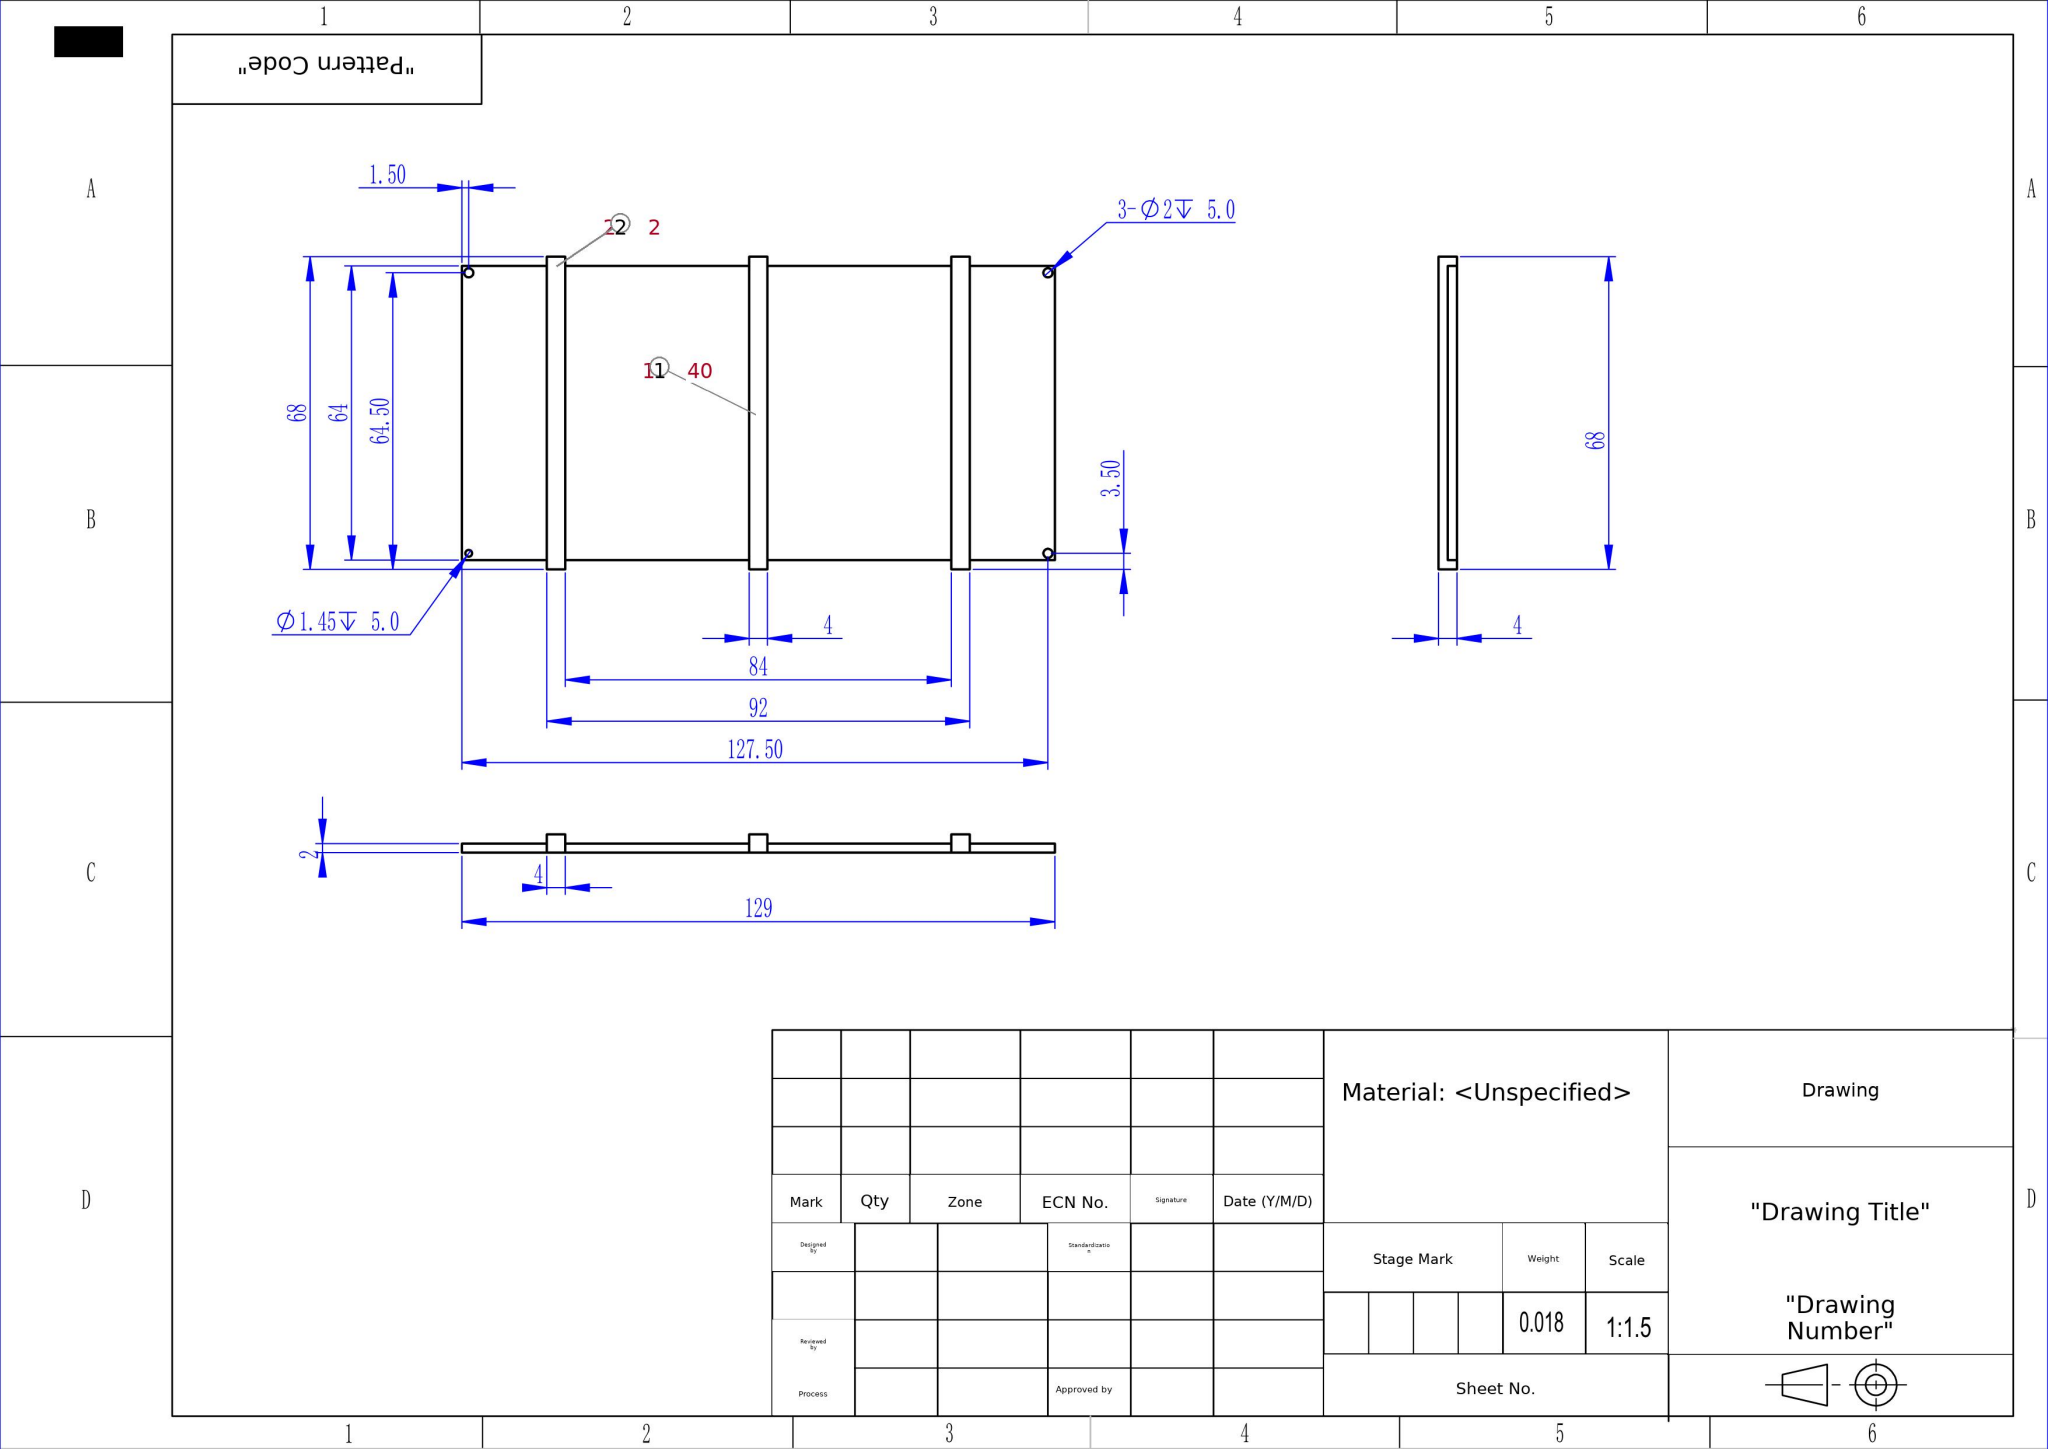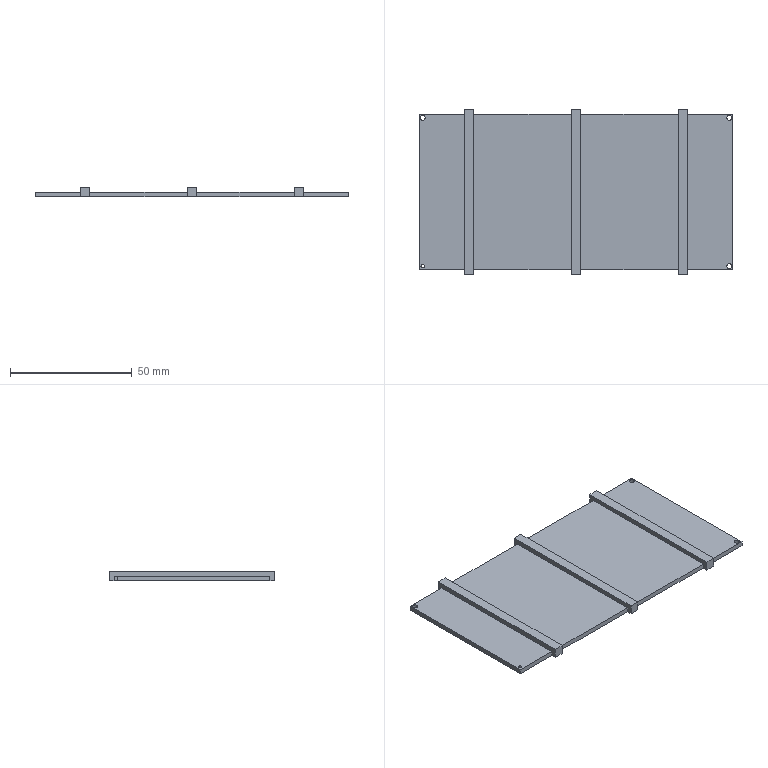Part | SolidWorks | mm | 1 solid | 38 faces | box 129 x 68 x 4 mm | volume 18218 mm3 | plane 30 | cylinder 8 | commonest cylinder face diameters 2 x6 1.45 x2
build123d program:
from build123d import *

# Parameters (mm, degrees)
BOSS_EXTRUDE1_DEPTH = 2
SKETCH2_W           = 4
SKETCH2_H           = 68
BOSS_EXTRUDE2_DEPTH = 2
SKETCH3_R           = 1
SKETCH3_R_2         = 0.725
CUT_EXTRUDE1_DEPTH  = 5


with BuildPart() as part:
    # Model → Boss-Extrude1 (new body)
    with BuildSketch(Plane.XY):
        Polygon((257.556, 185.18), (276.056, 185.18), (276.056, 187.18), (280.056, 187.18), (280.056, 185.18), (320.056, 185.18), (320.056, 187.18), (324.056, 187.18), (324.056, 185.18), (364.056, 185.18), (364.056, 187.18), (368.056, 187.18), (368.056, 185.18), (386.556, 185.18), (386.556, 173.18), (386.556, 169.18), (386.556, 137.18), (386.556, 133.18), (386.556, 121.18), (368.056, 121.18), (368.056, 119.18), (364.056, 119.18), (364.056, 121.18), (332.556, 121.18), (324.056, 121.18), (324.056, 119.18), (322.056, 119.18), (320.056, 119.18), (320.056, 121.18), (311.556, 121.18), (280.056, 121.18), (280.056, 119.18), (276.056, 119.18), (276.056, 121.18), (257.556, 121.18), (257.556, 133.18), (257.556, 137.18), (257.556, 169.18), (257.556, 173.18), align=None)
    extrude(amount=BOSS_EXTRUDE1_DEPTH)

    # Sketch2 → Boss-Extrude2 (add)
    with BuildSketch(Plane.XY.offset(2)):
        with Locations((366.056, 153.18)):
            Rectangle(SKETCH2_W, SKETCH2_H)
        with Locations((322.056, 153.18)):
            Rectangle(SKETCH2_W, SKETCH2_H)
        with Locations((278.056, 153.18)):
            Rectangle(SKETCH2_W, SKETCH2_H)
    extrude(amount=BOSS_EXTRUDE2_DEPTH)

    # Sketch3 → Cut-Extrude1 (cut)
    with BuildSketch(Plane.XY.offset(2)):
        with Locations((259.056, 183.68)):
            Circle(SKETCH3_R)
        with Locations((385.056, 183.68)):
            Circle(SKETCH3_R)
        with Locations((385.056, 122.68)):
            Circle(SKETCH3_R)
        with Locations((259.056, 122.68)):
            Circle(SKETCH3_R_2)
    extrude(amount=-CUT_EXTRUDE1_DEPTH, mode=Mode.SUBTRACT)


solid = part.part